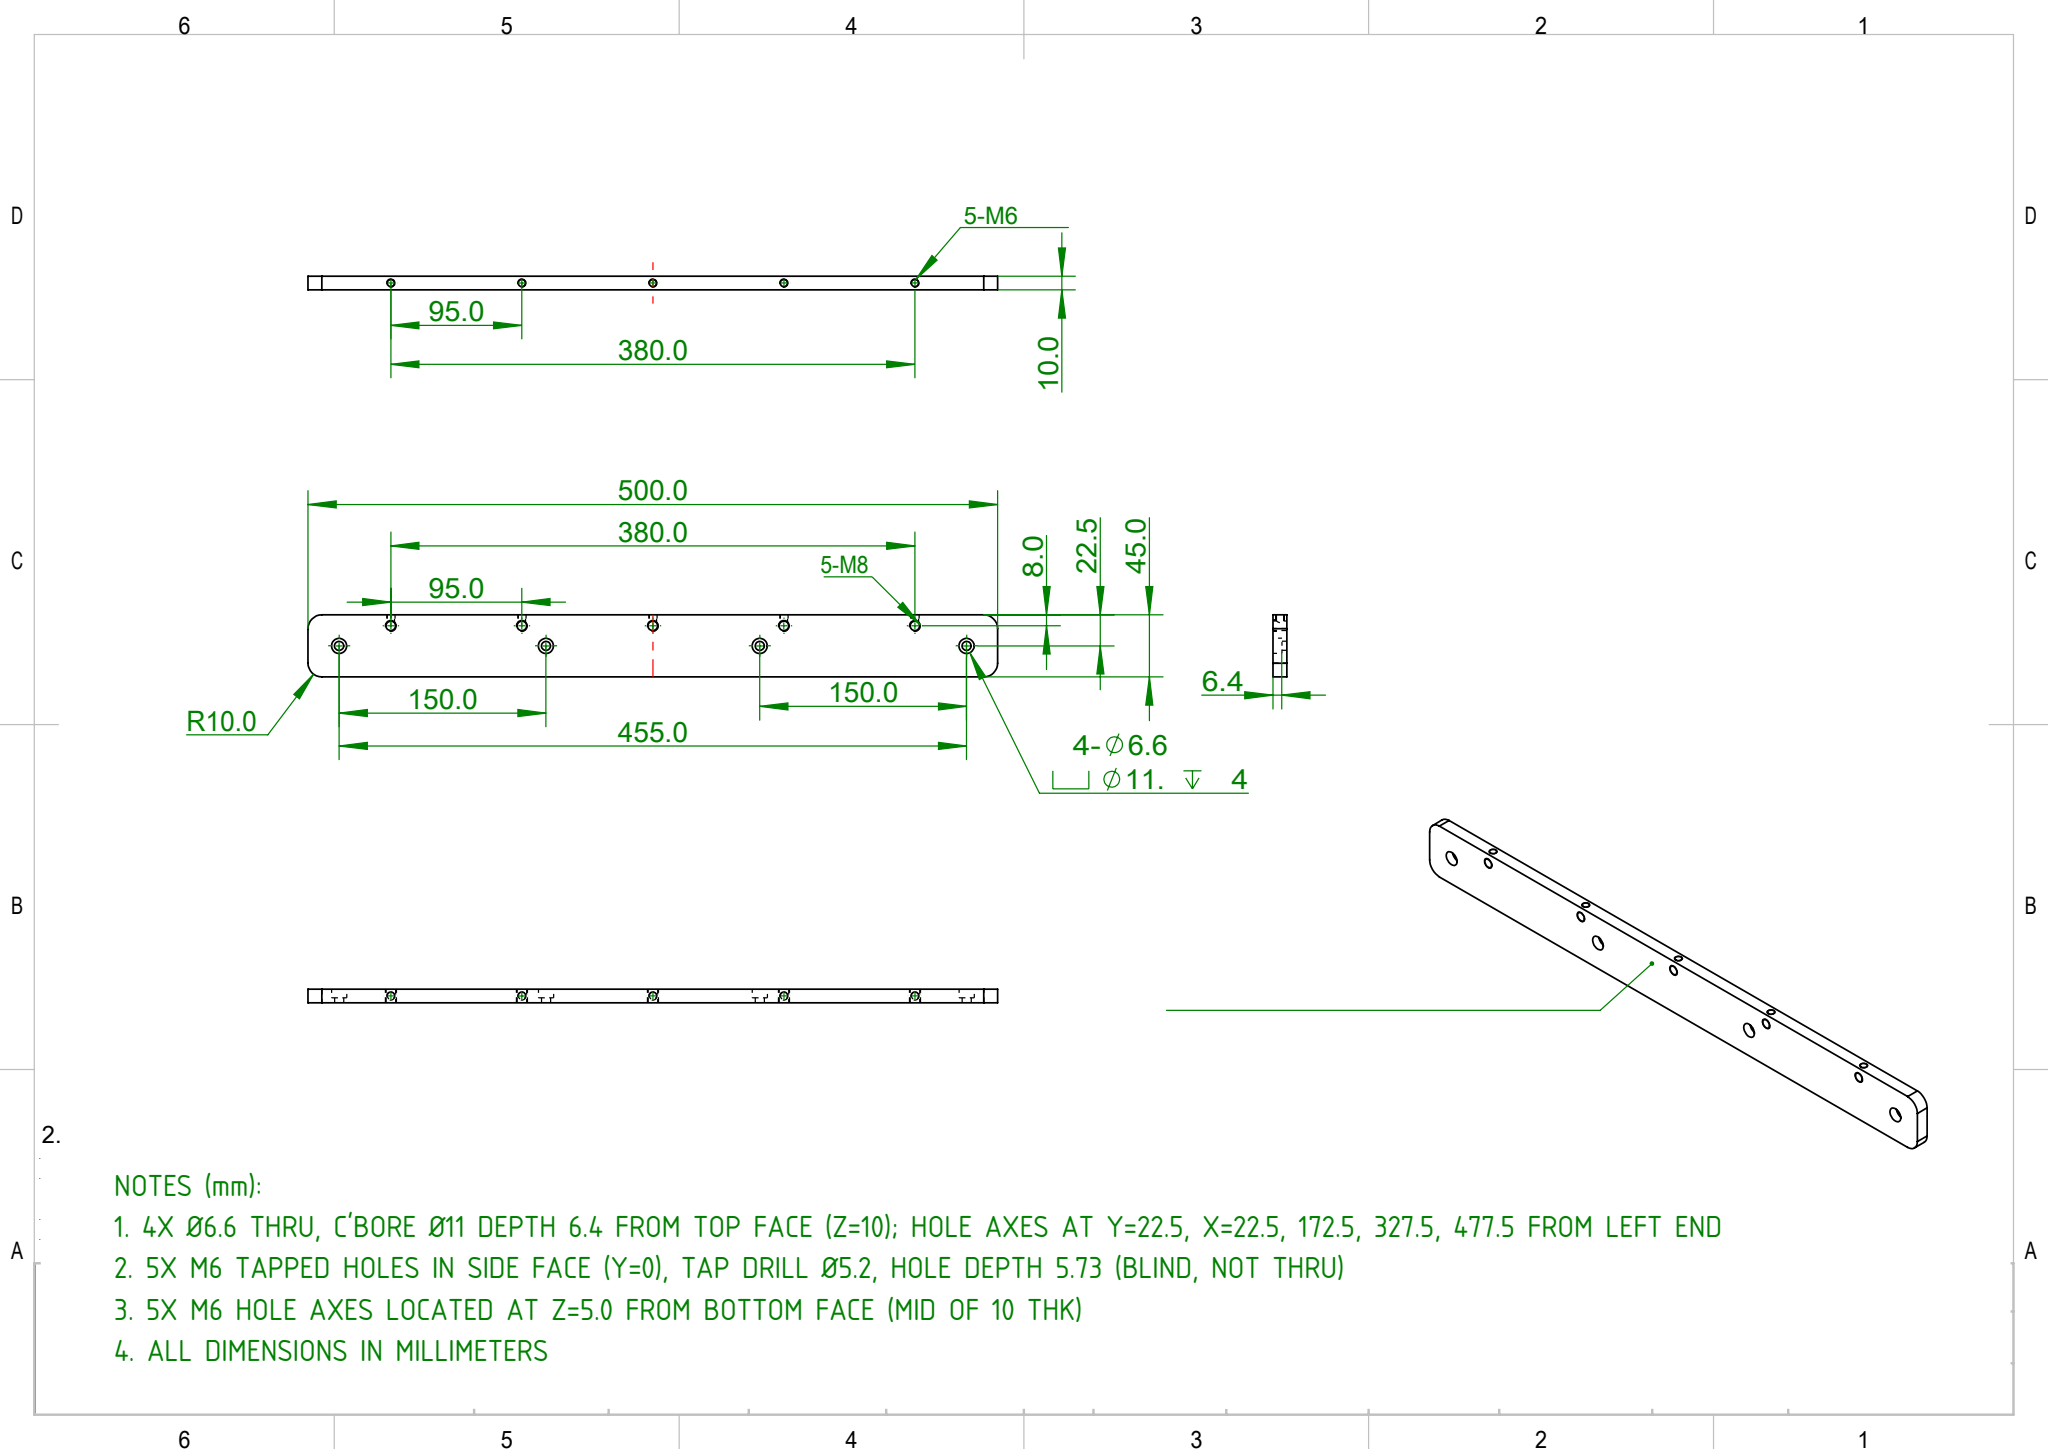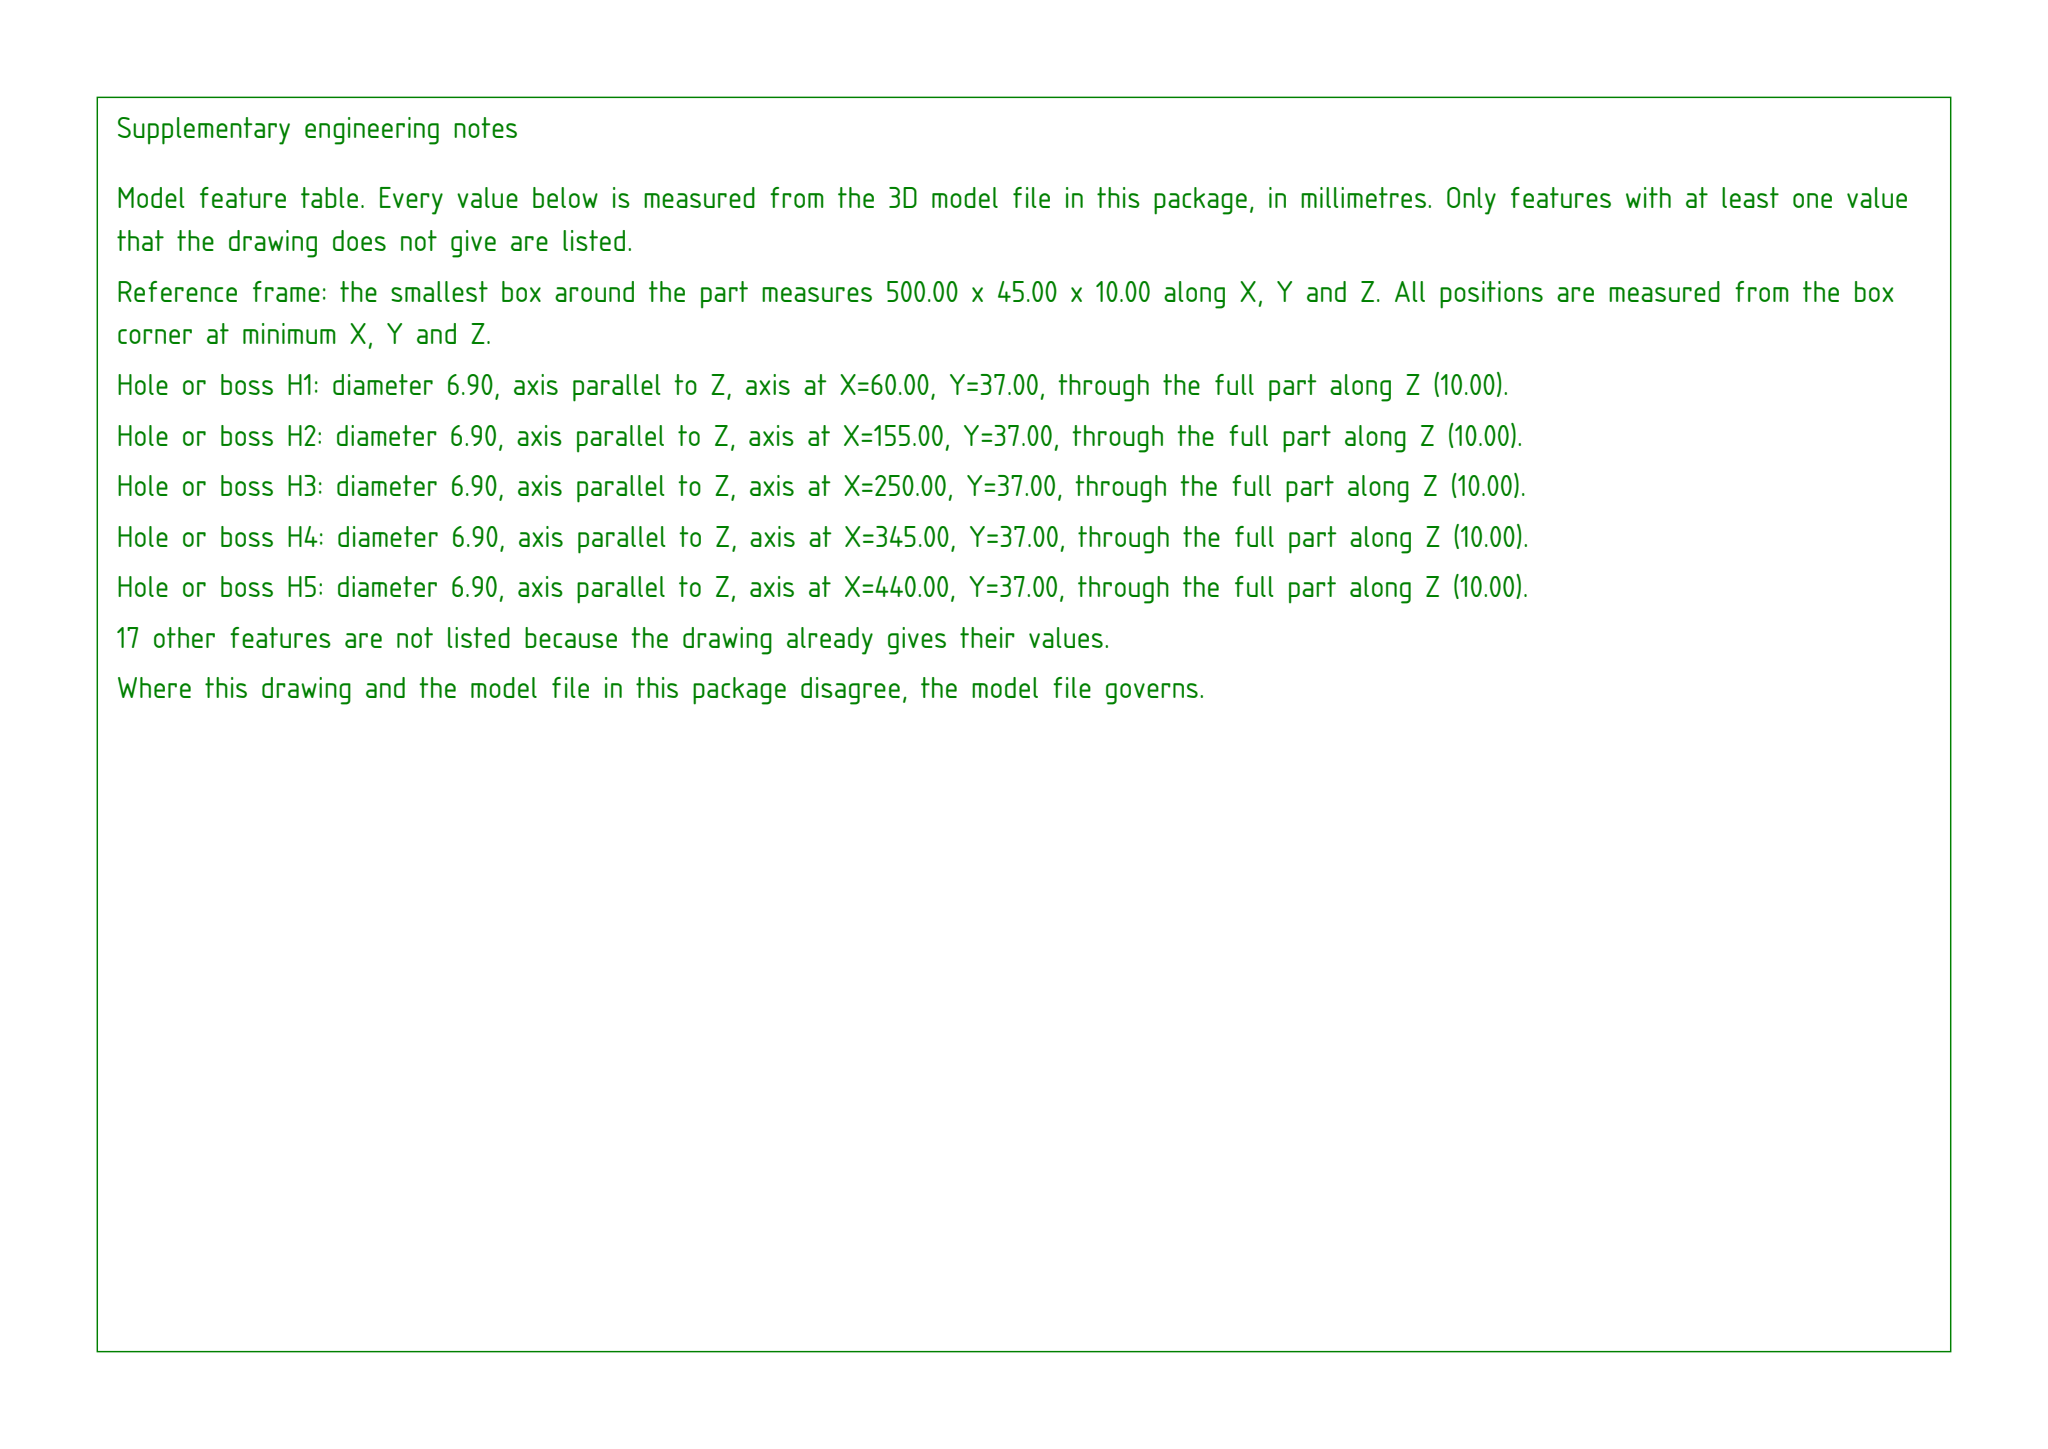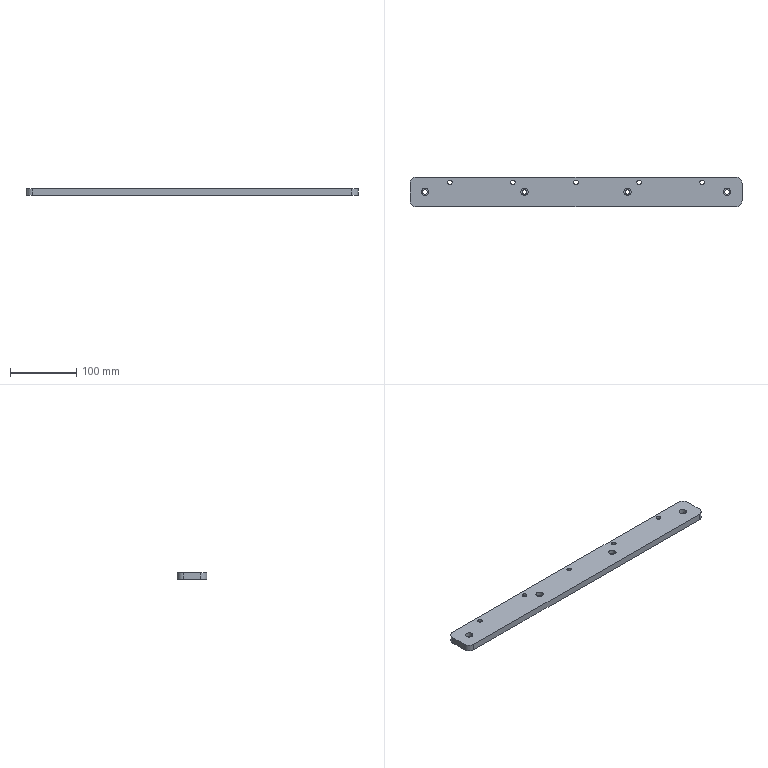Part | SolidWorks | mm | 1 solid | 50 faces | box 500 x 45 x 10 mm | volume 218835 mm3 | cylinder 40 | plane 10 | commonest cylinder face diameters 5.2 x10 6.9 x10 11 x8 6.6 x8 20 x4
Drawing notes:
4X Ø6.6 THRU, C'BORE Ø11 DEPTH 6.4 FROM TOP FACE (Z=10); HOLE AXES AT Y=22.5, X=22.5, 172.5, 327.5, 477.5 FROM LEFT END | from the solid: cylinders dia 6.6 axis z len 3.6 at (22.5,172.5,327.5,477.5; y=22.5) and dia 11.0 axis z len 6.4 at same xy; plate thickness bbox z=10
5X M6 TAPPED HOLES IN SIDE FACE (Y=0), TAP DRILL Ø5.2, HOLE DEPTH 5.73 (BLIND, NOT THRU) | from the solid: cylinders dia 5.2 axis y, length 5.73, at x=60,155,250,345,440
5X M6 HOLE AXES LOCATED AT Z=5.0 FROM BOTTOM FACE (MID OF 10 THK) | from the solid: cylinders dia 5.2 axis y, pos_other_axes z=5.0; bbox z=10.0
ALL DIMENSIONS IN MILLIMETERS | from the solid: STEP model facts stated in mm
build123d program:
from build123d import *

# Parameters (mm, degrees)
SKETCH1_W                                       = 500
SKETCH1_H                                       = 45
BOSS_EXTRUDE1_DEPTH                             = 5
SKETCH4_R                                       = 3.45
CUT_EXTRUDE1_DEPTH                              = 10
SKETCH8_R                                       = 2.6
CUT_EXTRUDE2_DEPTH                              = 10
LPATTERN1_COUNT                                 = 5
LPATTERN1_PITCH                                 = 95
FILLET1_R                                       = 10
M6_HEX_SOCKET_HEAD_CAP_SCREW_CBORE1_D           = 6.6
M6_HEX_SOCKET_HEAD_CAP_SCREW_CBORE1_CBORE_D     = 11
M6_HEX_SOCKET_HEAD_CAP_SCREW_CBORE1_CBORE_DEPTH = 6.4


with BuildPart() as part:
    # Sketch1 → Boss-Extrude1 (new, symmetric)
    with BuildSketch(Plane.XY):
        Rectangle(SKETCH1_W, SKETCH1_H)
    extrude(amount=BOSS_EXTRUDE1_DEPTH, both=True)

    # Sketch4 → Cut-Extrude1 (cut)
    with BuildSketch(Plane.XY.offset(5)):
        with Locations((-190, 14.5)):
            Circle(SKETCH4_R)
    cut_extrude1 = extrude(amount=-CUT_EXTRUDE1_DEPTH, mode=Mode.SUBTRACT)

    # Sketch8 → Cut-Extrude2 (cut)
    with BuildSketch(Plane(origin=(0, 22.5, 0), x_dir=(1, 0, 0), z_dir=(0, 1, 0))):
        with Locations(Location((-190, 0, 0), (0, 0, 270))):
            Circle(SKETCH8_R)
    cut_extrude2 = extrude(amount=-CUT_EXTRUDE2_DEPTH, mode=Mode.SUBTRACT)

    # LPattern1: Cut-Extrude1, Cut-Extrude2 ×5
    with Locations(*[(i * LPATTERN1_PITCH, 0, 0) for i in range(1, LPATTERN1_COUNT)]):
        add(cut_extrude1, mode=Mode.SUBTRACT)
        add(cut_extrude2, mode=Mode.SUBTRACT)

    # Fillet1
    fillet1_edges = [part.edges().sort_by_distance(p)[0] for p in [
        (250, -22.5, 0),
        (-250, -22.5, 0),
        (-250, 22.5, 0),
        (250, 22.5, 0),
    ]]
    fillet(fillet1_edges, radius=FILLET1_R)

    # M6 Hex Socket Head Cap Screw CBORE1 (through all)
    with Locations(Plane(origin=(-227.5, 0, 5), x_dir=(1, 0, 0), z_dir=(0, 0, 1))):
        with Locations((0, 0), (150, 0), (305, 0), (455, 0)):
            CounterBoreHole(M6_HEX_SOCKET_HEAD_CAP_SCREW_CBORE1_D / 2, M6_HEX_SOCKET_HEAD_CAP_SCREW_CBORE1_CBORE_D / 2, M6_HEX_SOCKET_HEAD_CAP_SCREW_CBORE1_CBORE_DEPTH)


solid = part.part